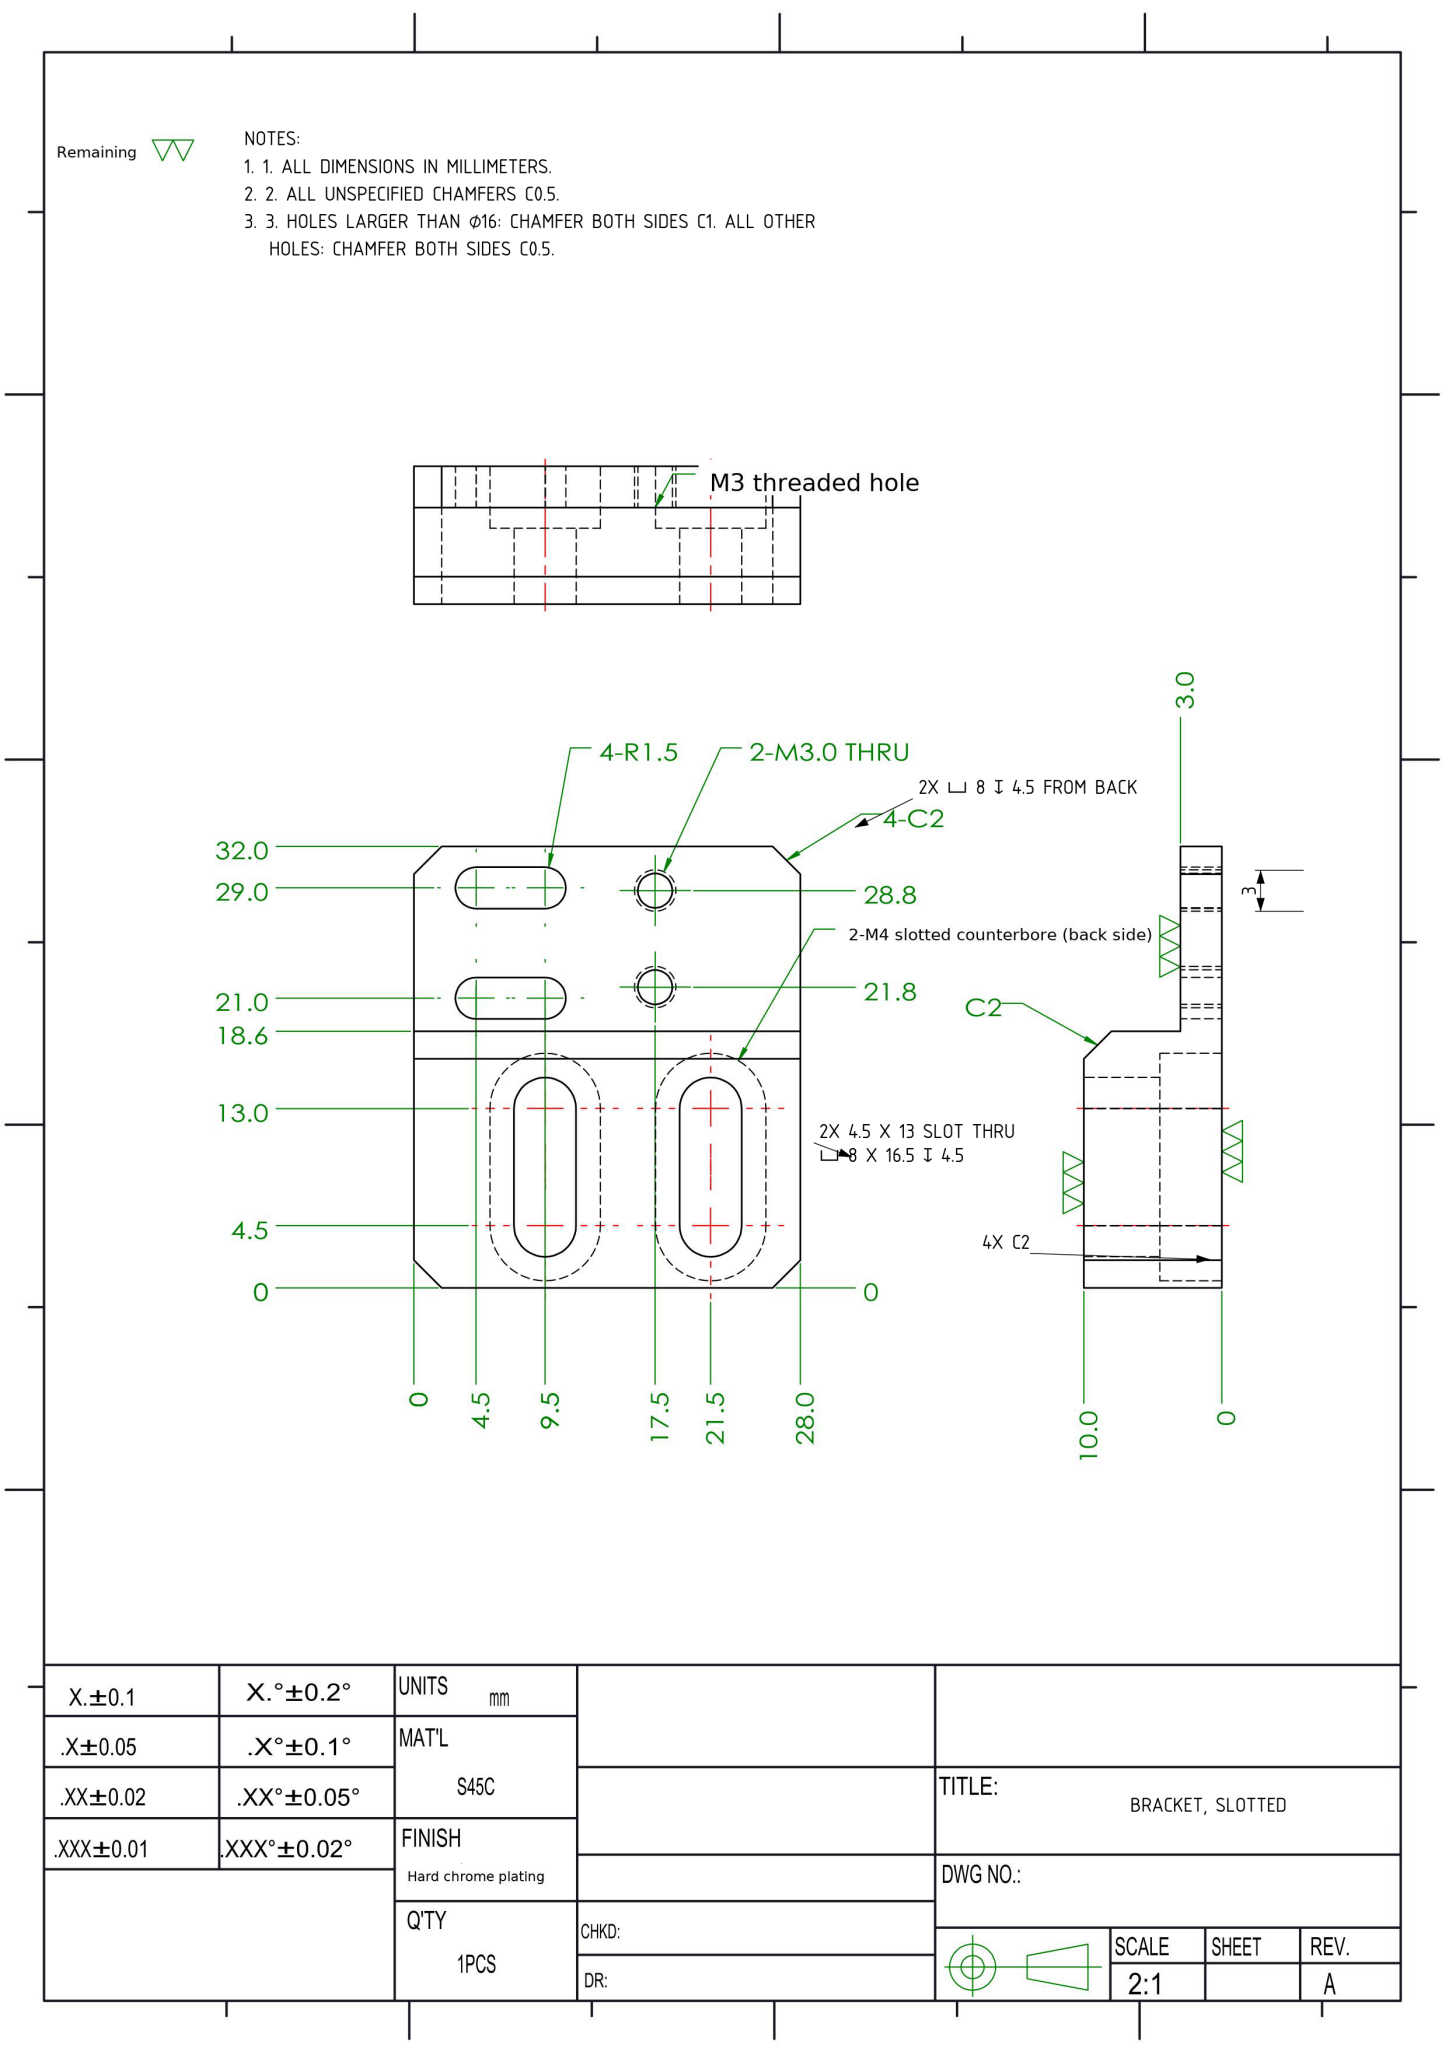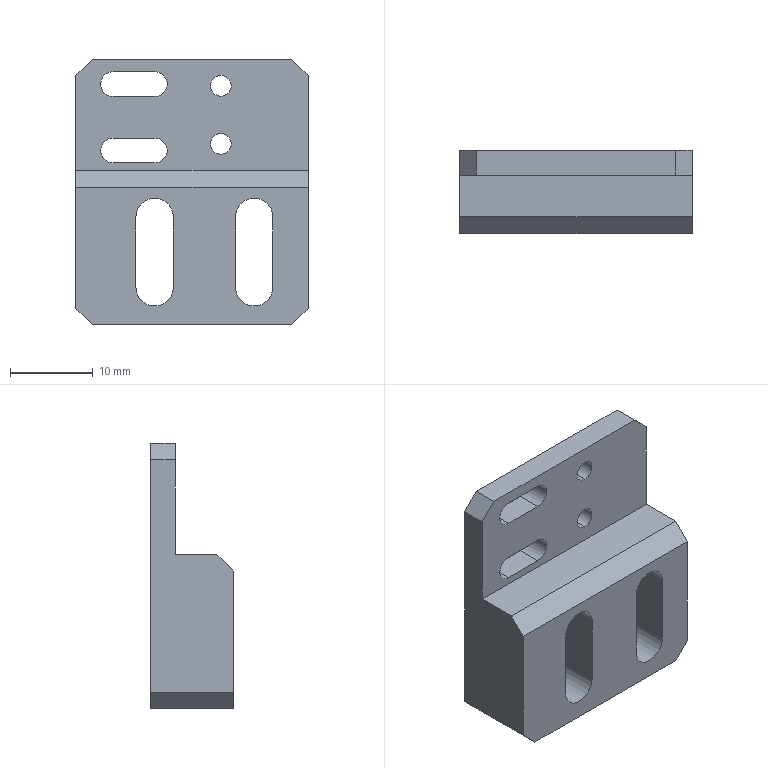Part | NX | mm | 1 solid | 47 faces | box 28 x 10 x 32 mm | volume 4402 mm3 | plane 27 | cylinder 20 | commonest cylinder face diameters 8 x6 4.5 x6 2.5 x4 3 x4